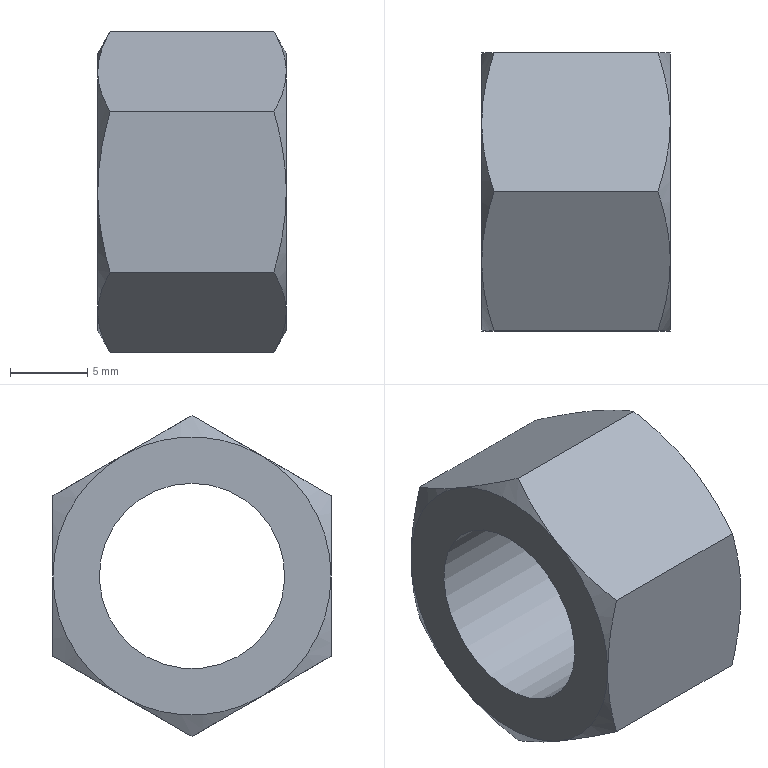Component | NX | NUT_M12 | 1 solid | 21 faces | volume 2031 mm3 | cone 12 | plane 8 | cylinder 1 | commonest cylinder face diameters 12 x1